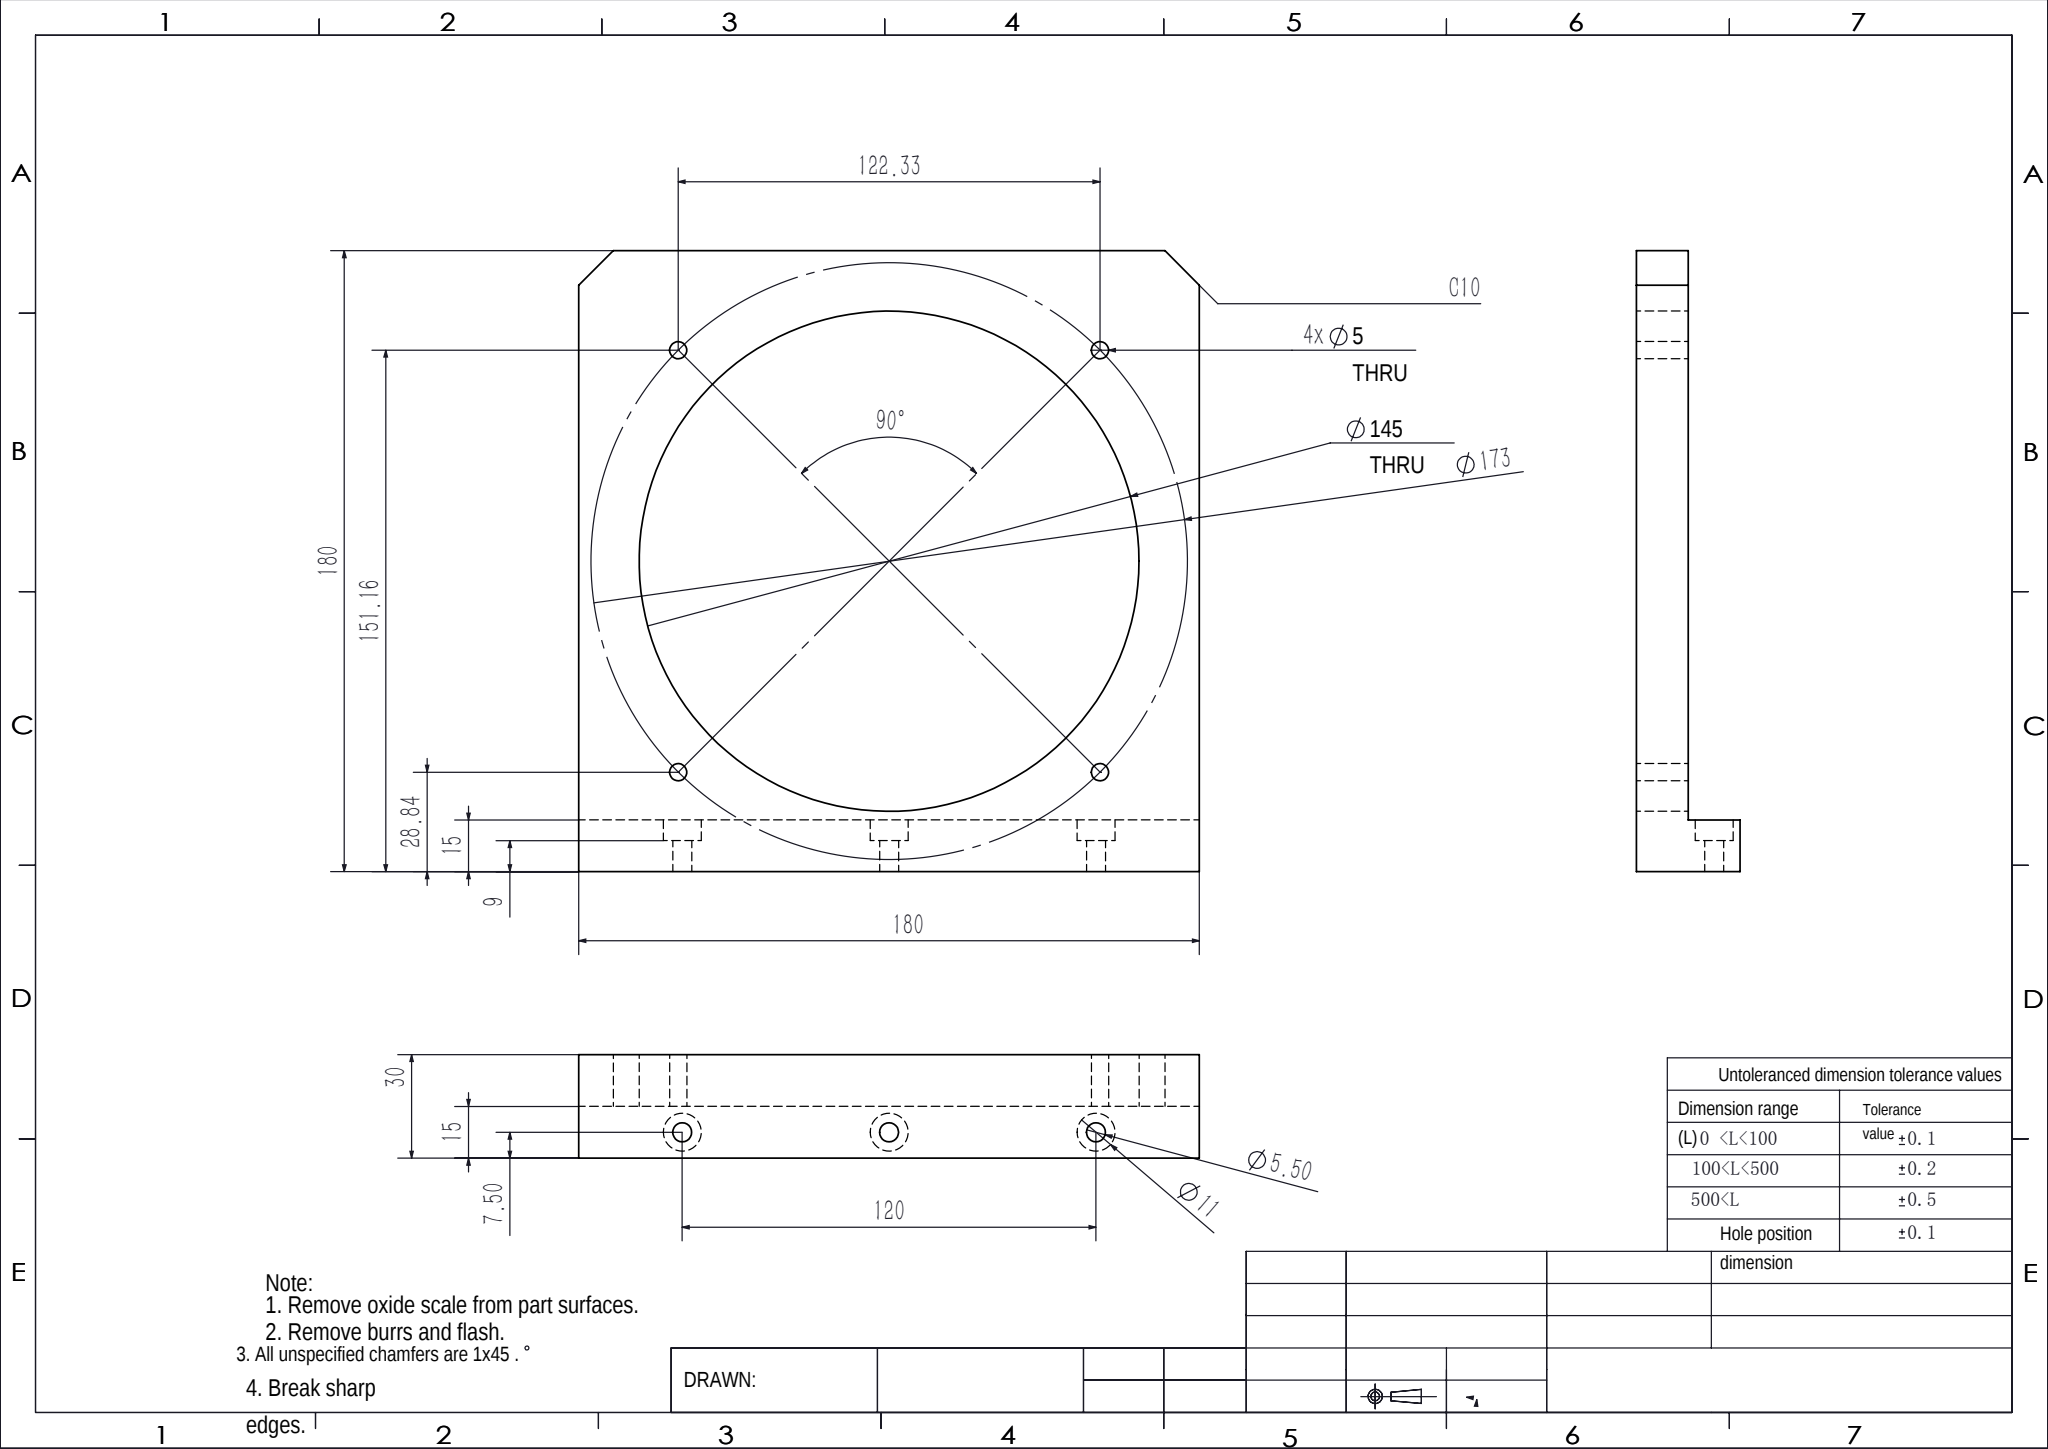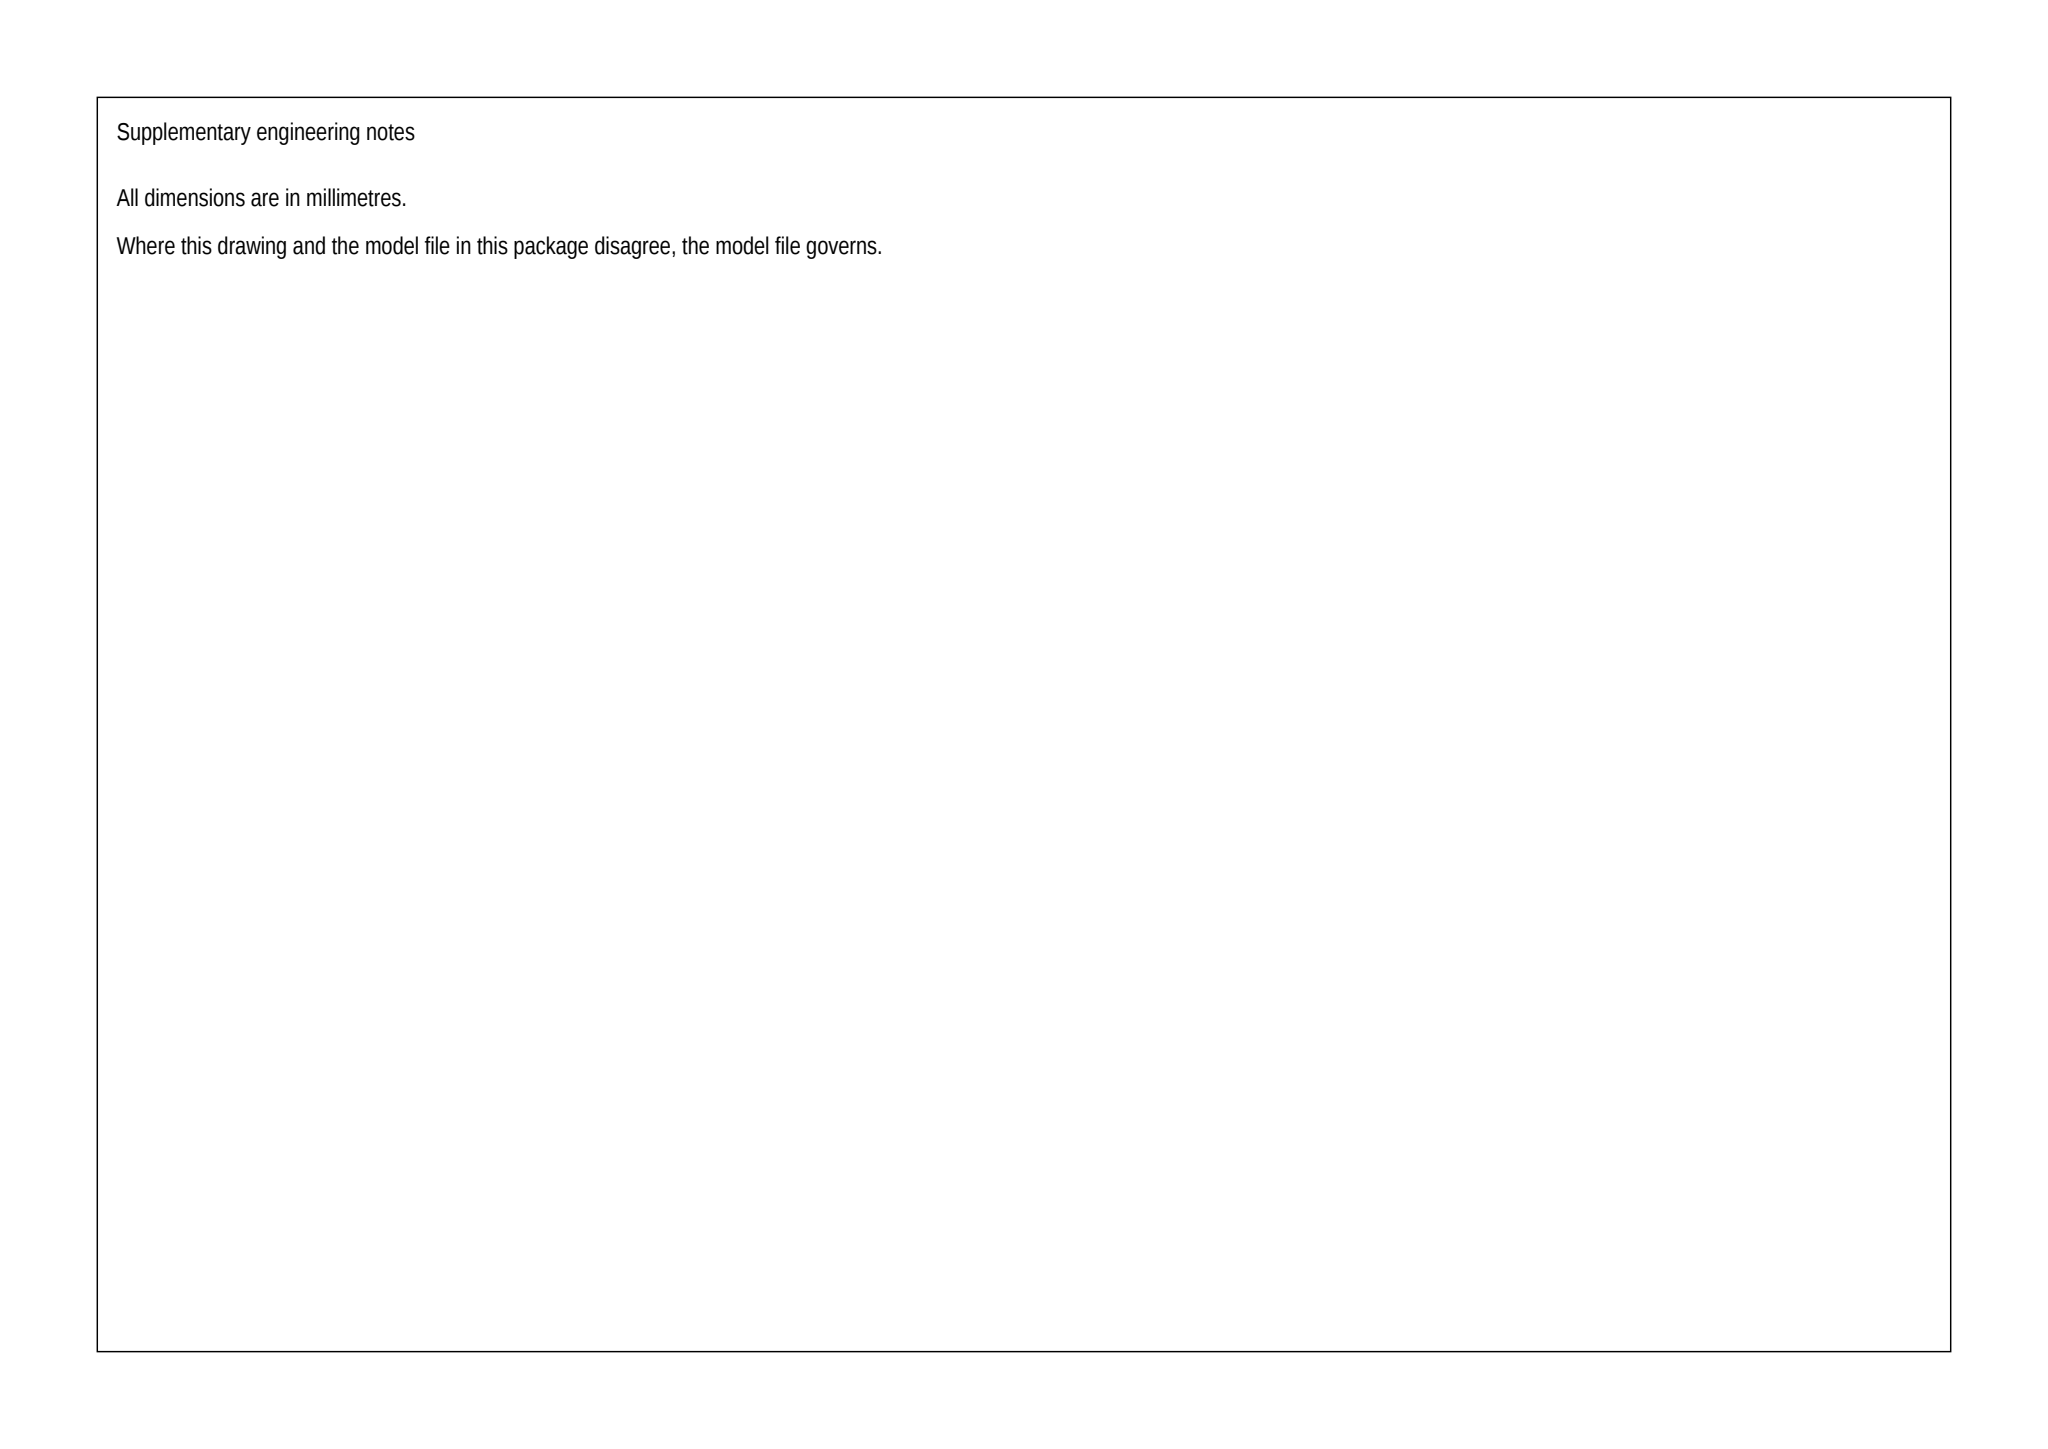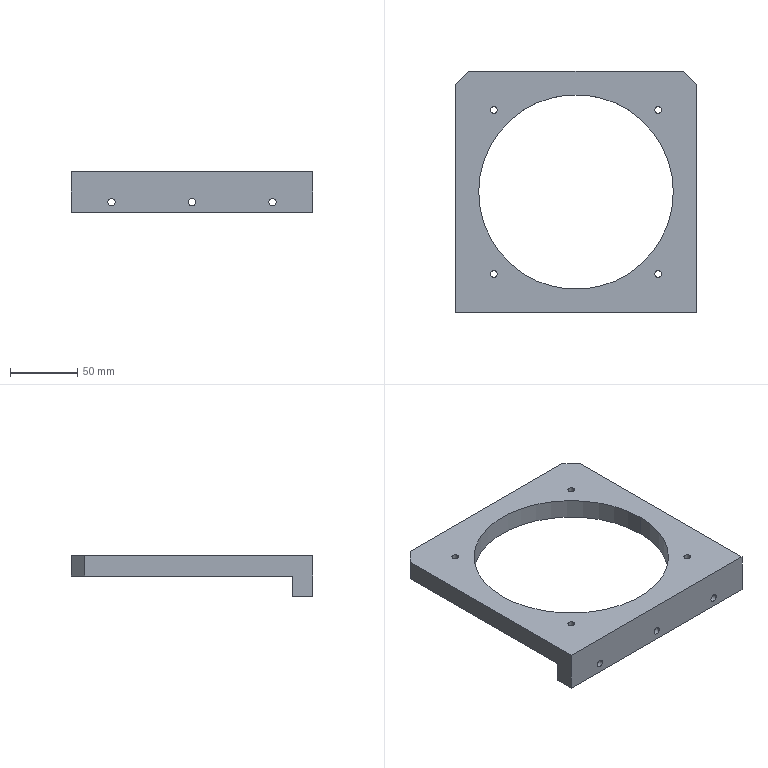Part | SolidWorks | mm | 1 solid | 35 faces | box 180 x 180 x 30 mm | volume 273775 mm3 | cylinder 22 | plane 13 | commonest cylinder face diameters 5 x8 11 x6 5.5 x6 145 x2
build123d program:
from build123d import *

# Parameters (mm, degrees)
SKETCH1_W           = 180
SKETCH1_H           = 180
BOSS_EXTRUDE1_DEPTH = 15
SKETCH2_W           = 180
SKETCH2_H           = 15
BOSS_EXTRUDE2_DEPTH = 15
SKETCH4_R           = 72.5
CUT_EXTRUDE1_DEPTH  = 131.767
CHAMFER2_SIZE       = 10
SKETCH7_R           = 2.75
CUT_EXTRUDE2_DEPTH  = 189.547
SKETCH8_R           = 5.5
CUT_EXTRUDE3_DEPTH  = 6
SKETCH9_R           = 2.5
CUT_EXTRUDE4_DEPTH  = 129.16


with BuildPart() as part:
    # Sketch1 → Boss-Extrude1 (new body)
    with BuildSketch(Plane.XY):
        Rectangle(SKETCH1_W, SKETCH1_H)
    extrude(amount=BOSS_EXTRUDE1_DEPTH)

    # Sketch2 → Boss-Extrude2 (add)
    with BuildSketch(Plane(origin=(0, 0, 0), x_dir=(-1, 0, 0), z_dir=(0, 0, -1))):
        with Locations((0, -82.5)):
            Rectangle(SKETCH2_W, SKETCH2_H)
    extrude(amount=BOSS_EXTRUDE2_DEPTH)

    # Sketch4 → Cut-Extrude1 (cut, through all)
    with BuildSketch(Plane.XY.offset(15)):
        Circle(SKETCH4_R)
    extrude(amount=-CUT_EXTRUDE1_DEPTH, mode=Mode.SUBTRACT)

    # Chamfer2
    chamfer2_edges = [part.edges().sort_by_distance(p)[0] for p in [
        (-90, 90, 7.5),
        (90, 90, 7.5),
    ]]
    chamfer(chamfer2_edges, length=CHAMFER2_SIZE)

    # Sketch7 → Cut-Extrude2 (cut, through all)
    with BuildSketch(Plane(origin=(0, -75, 0), x_dir=(1, 0, 0), z_dir=(0, 1, 0))):
        with Locations(Location((-60, 7.5, 0), (0, 0, 180))):
            Circle(SKETCH7_R)
        with Locations(Location((60, 7.5, 0), (0, 0, 180))):
            Circle(SKETCH7_R)
        with Locations(Location((0, 7.5, 0), (0, 0, 180))):
            Circle(SKETCH7_R)
    extrude(amount=-CUT_EXTRUDE2_DEPTH, mode=Mode.SUBTRACT)

    # Sketch8 → Cut-Extrude3 (cut)
    with BuildSketch(Plane(origin=(0, -75, 0), x_dir=(1, 0, 0), z_dir=(0, 1, 0))):
        with Locations(Location((-60, 7.5, 0), (0, 0, 180))):
            Circle(SKETCH8_R)
        with Locations(Location((0, 7.5, 0), (0, 0, 180))):
            Circle(SKETCH8_R)
        with Locations(Location((60, 7.5, 0), (0, 0, 180))):
            Circle(SKETCH8_R)
    extrude(amount=-CUT_EXTRUDE3_DEPTH, mode=Mode.SUBTRACT)

    # Sketch9 → Cut-Extrude4 (cut, through all)
    with BuildSketch(Plane(origin=(0, 0, 0), x_dir=(-1, 0, 0), z_dir=(0, 0, -1))):
        with Locations((-61.165, 61.165)):
            Circle(SKETCH9_R)
        with Locations((61.165, 61.165)):
            Circle(SKETCH9_R)
        with Locations((61.165, -61.165)):
            Circle(SKETCH9_R)
        with Locations((-61.165, -61.165)):
            Circle(SKETCH9_R)
    extrude(amount=-CUT_EXTRUDE4_DEPTH, mode=Mode.SUBTRACT)


solid = part.part